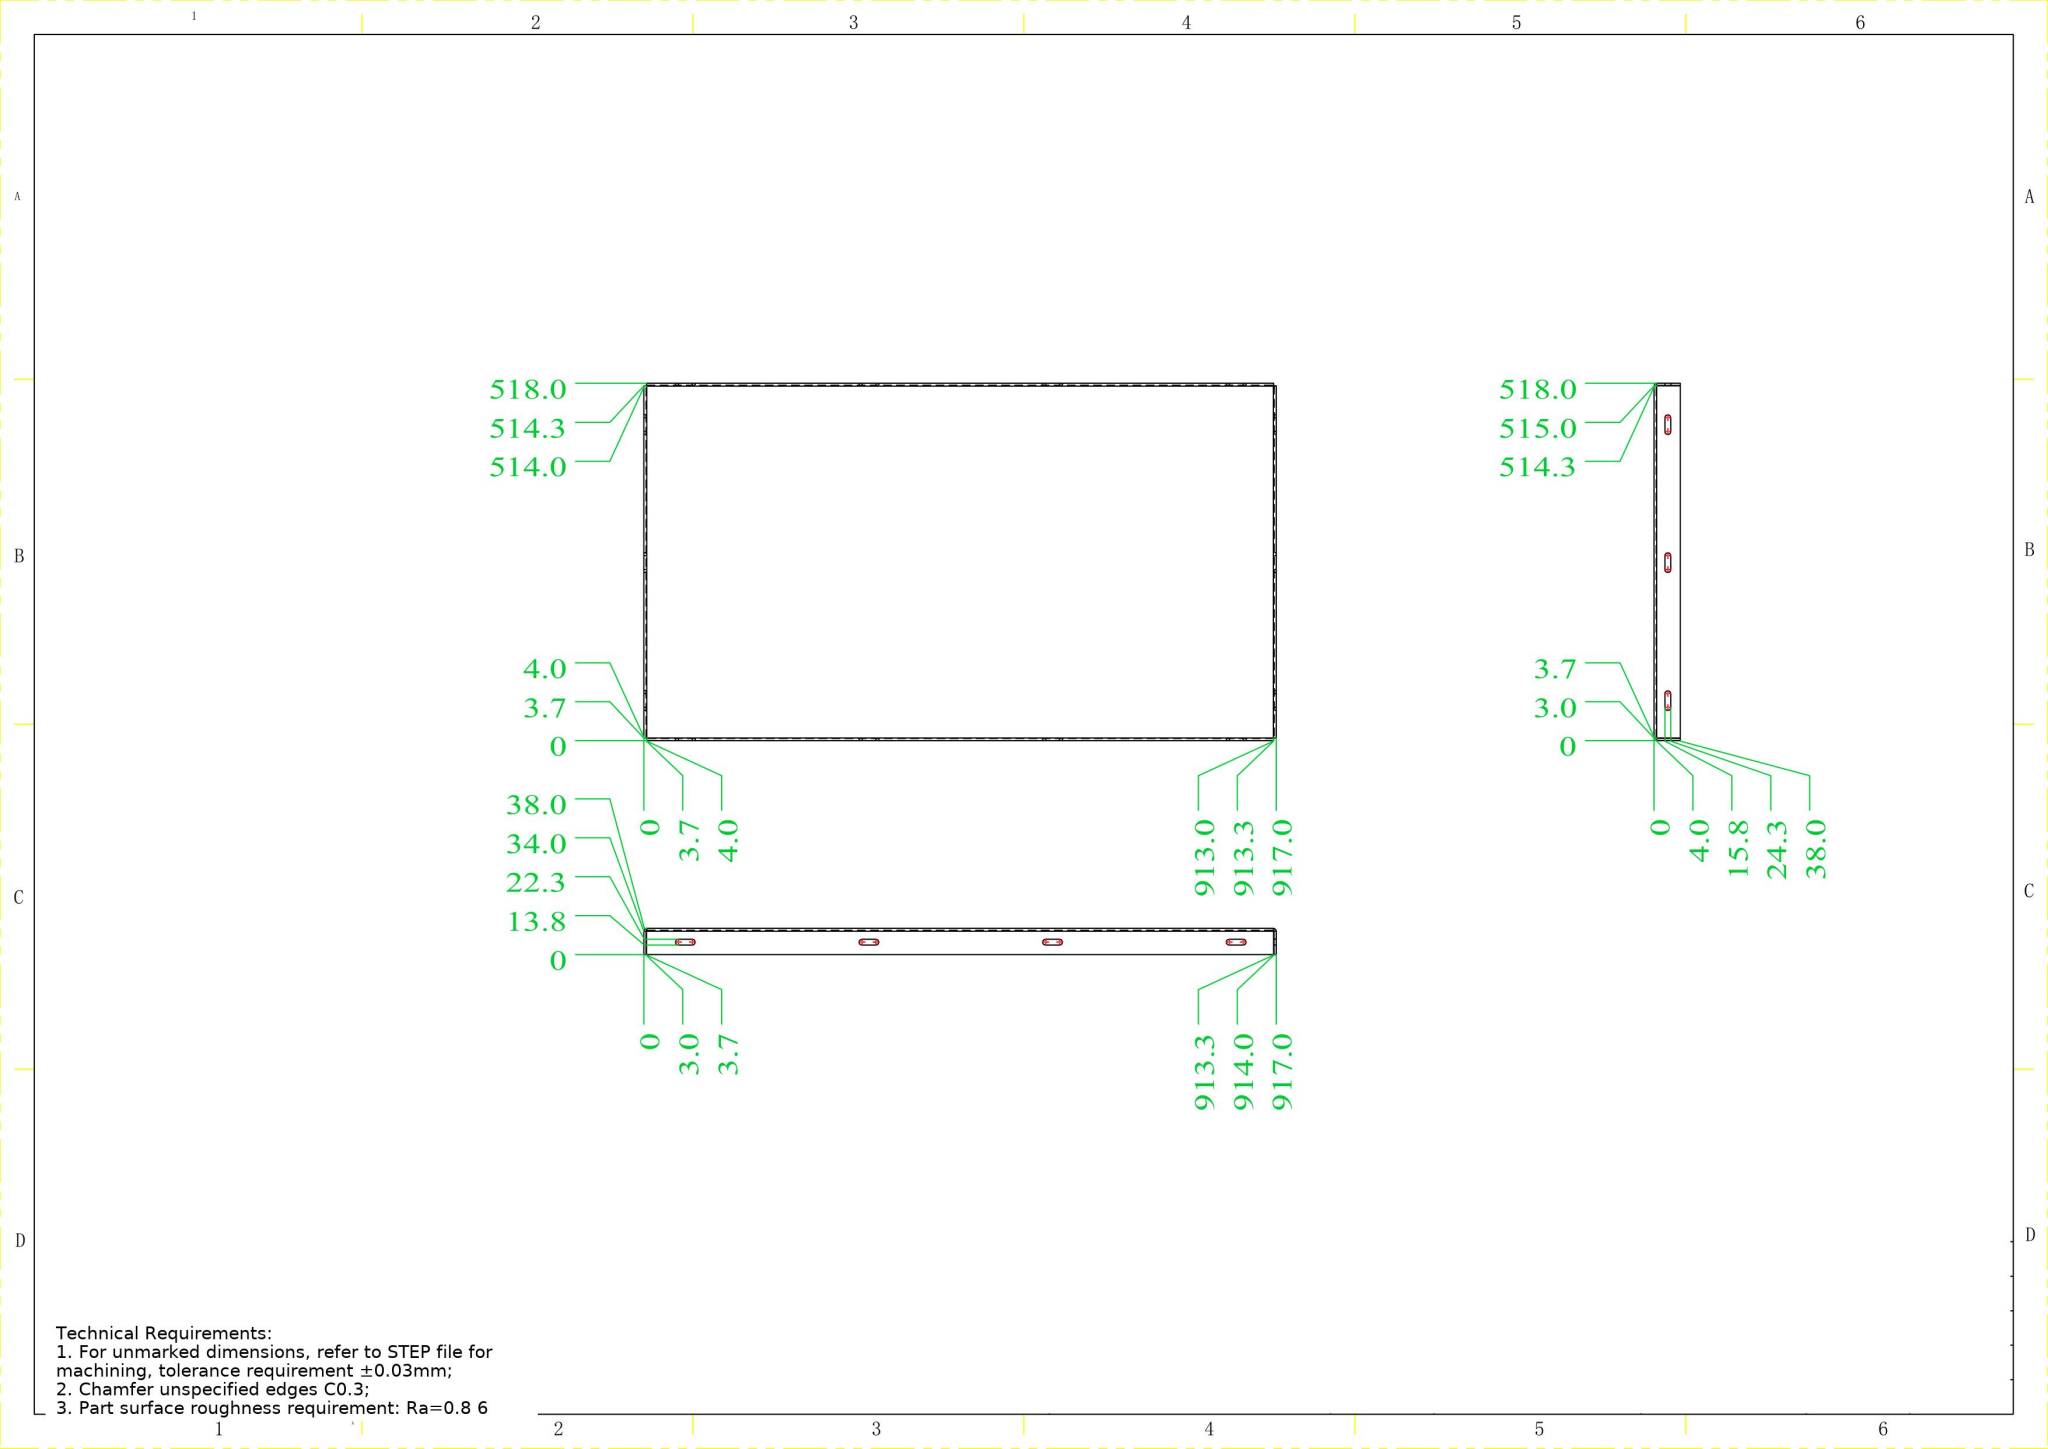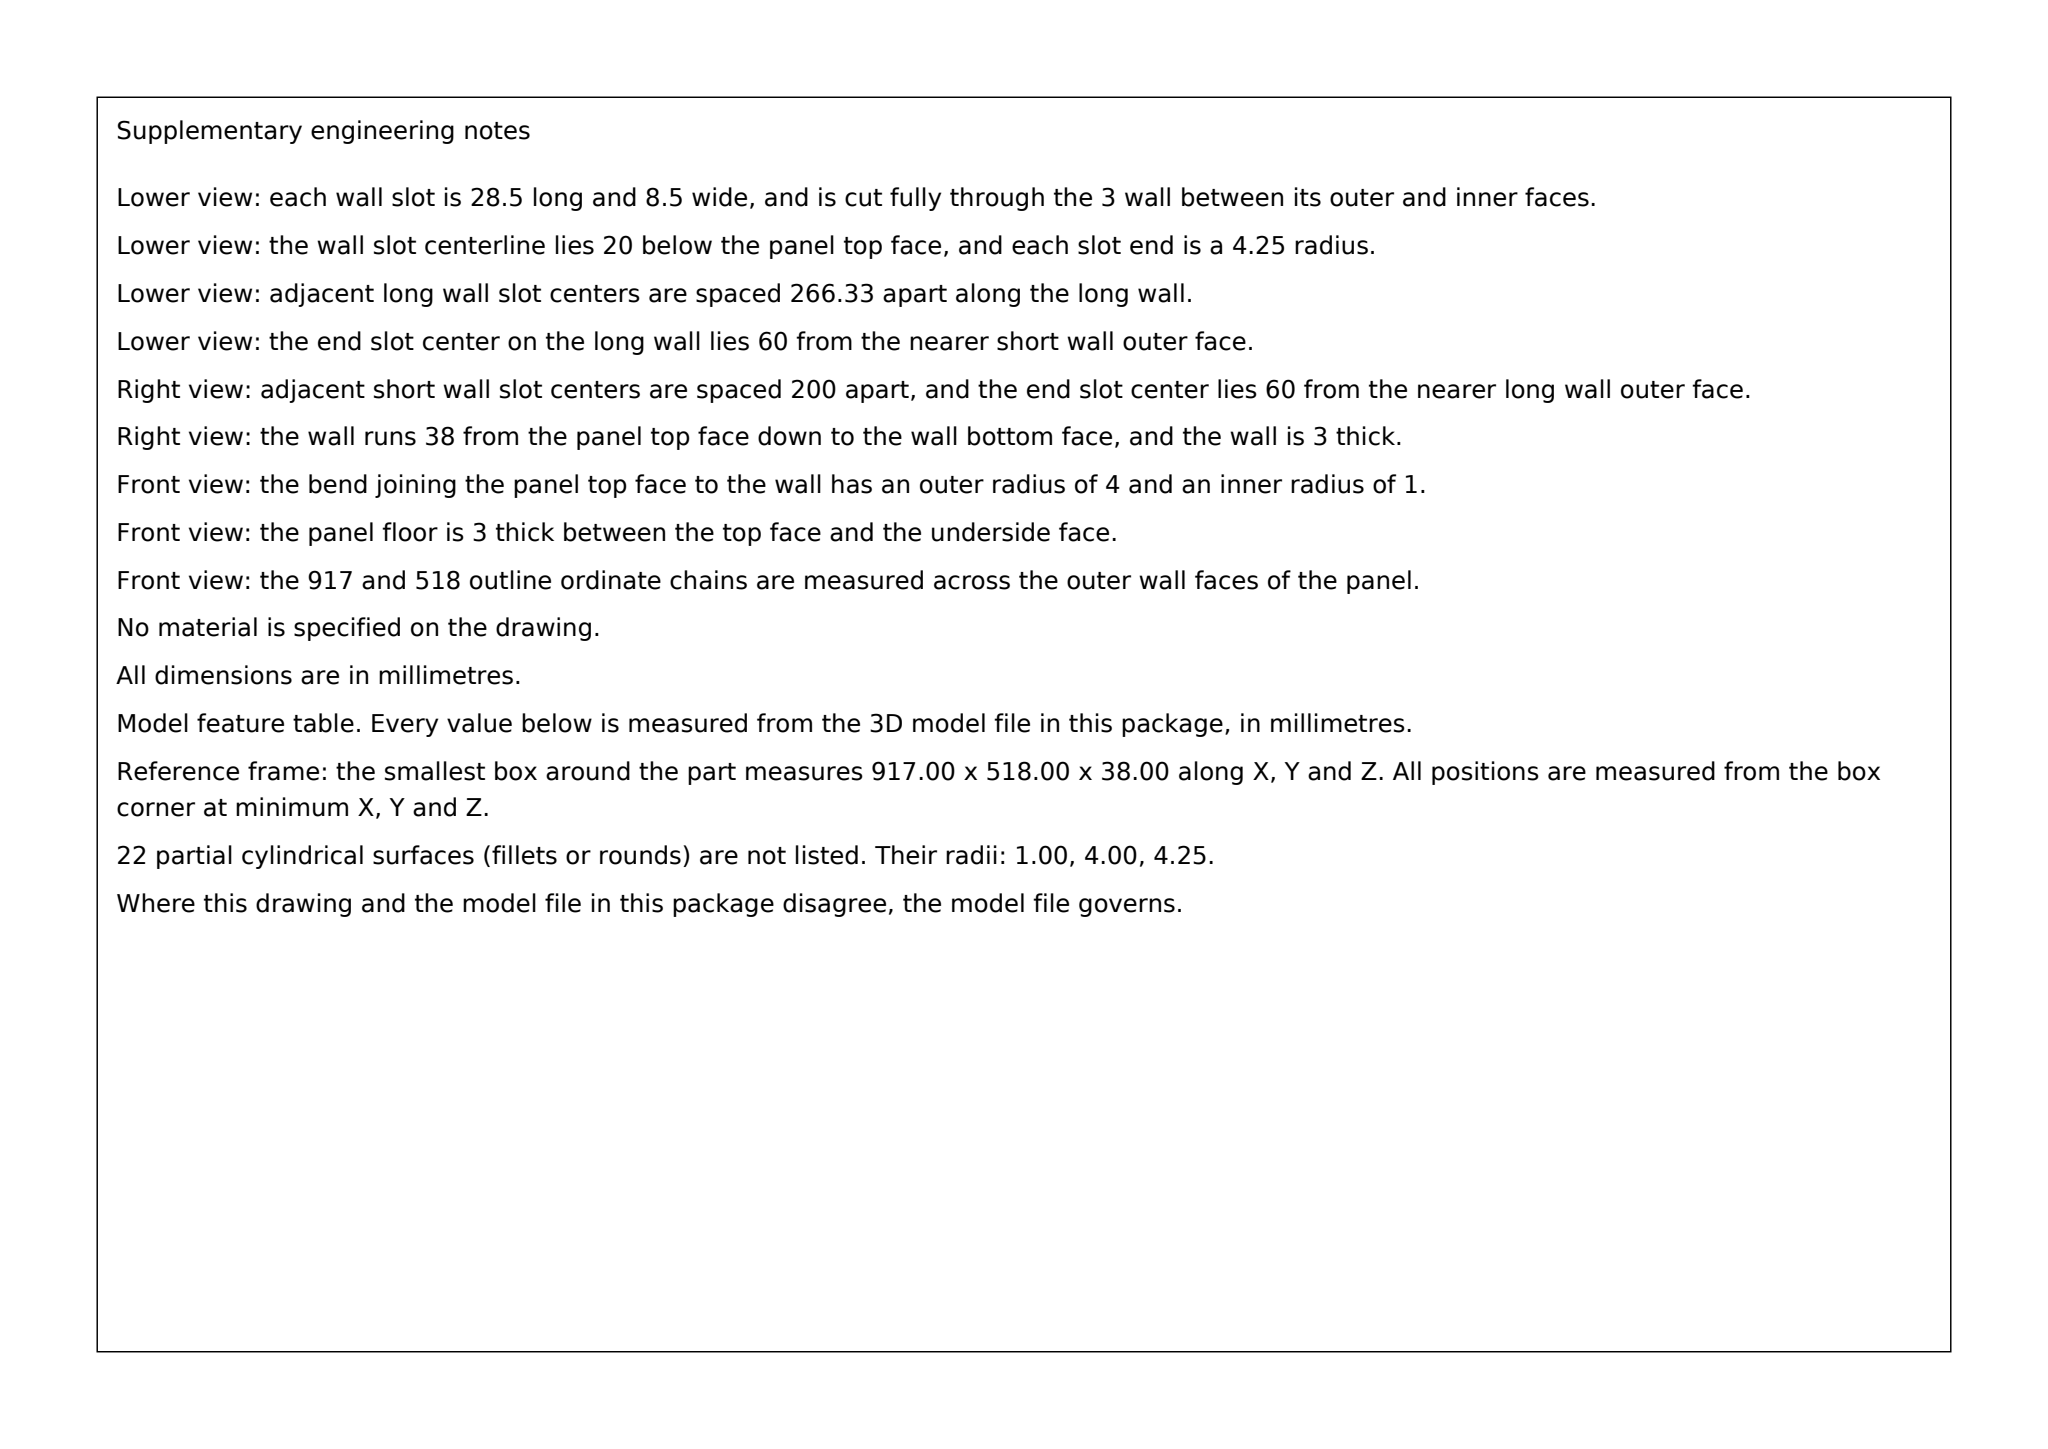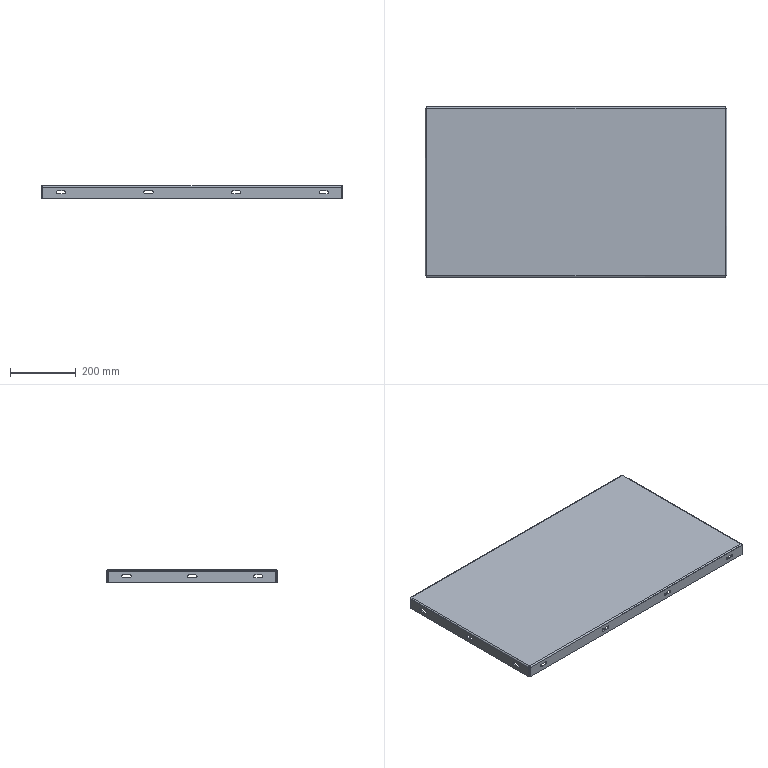Part | SolidWorks | mm | 1 solid | 94 faces | box 917 x 518 x 38 mm | volume 1704410 mm3 | plane 50 | cylinder 36 | spline 8 | commonest cylinder face diameters 8.5 x28 8 x4 2 x4
Drawing notes:
14X 8.5 WIDE OBROUND SLOT, 28.5 OVERALL LENGTH (20.0 BETWEEN END-RADII CENTERS), THRU 3.0 WALL, SLOT CENTERLINE AT Z=18.0 FROM BOTTOM FACE | from the solid: cylinders dia 8.5, length 3.0, pos z=18.0; paired centers 20 mm apart (e.g. y=48.03 & 68.03; x=50.03 & 70.03)
SLOTS IN EACH 917 LONG WALL (8 PLACES, 4 PER WALL): END-RADII CENTERS AT X=50.0 & 70.0, 316.4 & 336.4, 582.7 & 602.7, 849.0 & 869.0 FROM X=0 DATUM | from the solid: cylinders[8.5,"y",[50.03/70.03/316.36/336.36/582.69/602.69/849.02/869.02,null,18.0],3.0,2]
SLOTS IN EACH 518 END WALL (6 PLACES, 3 PER WALL): END-RADII CENTERS AT Y=48.0 & 68.0, 248.0 & 268.0, 448.0 & 468.0 FROM Y=0 DATUM | from the solid: cylinders[8.5,"x",[null,48.03/68.03/248.03/268.03/448.03/468.03,18.0],3.0,2]
PATTERN: 4X SLOTS TYP EACH 917 SIDE, 3X SLOTS TYP EACH 518 SIDE, 14 SLOTS TOTAL | from the solid: cylinders dia 8.5 axis y: 8 pair-entries count 2 (4 slots x 2 walls); axis x: 6 pair-entries count 2 (3 slots x 2 walls)
Ø8 INTERNAL LONGITUDINAL BORE AT Z=34.0, AXIS 4.0 FROM OUTSIDE FACE: 2X 909.6 LONG ALONG THE 917 EDGES (Y=4.0 AND Y=514.0), 2X 510.6 LONG ALONG THE 518 EDGES (X=4.0 AND X=913.0) | from the solid: cylinders[8.0,"x",[null,4.03/514.03,34.0],909.59] and cylinders[8.0,"y",[4.03/913.03,null,34.0],510.59]
Ø2 OPENING SLIT INTO EACH Ø8 LONGITUDINAL BORE, COAXIAL AT Z=34.0 AND 4.0 FROM OUTSIDE FACE, 4 PLACES, SAME LENGTHS AS BORES (909.6 / 510.6) | from the solid: cylinders[2.0,"x",[null,4.03/514.03,34.0],909.59] and cylinders[2.0,"y",[4.03/913.03,null,34.0],510.59]
STEP AT TOP OF WALLS: FACE AT Z=35.0, 3.0 BELOW THE Z=38.0 TOP FACE (38.0 OVERALL HEIGHT FROM Z=0 BOTTOM DATUM); STEP FACE BOUNDED BY X=3.0 TO 914.0 AND Y=3.0 TO 515.0 FROM X=0 / Y=0 DATUMS | from the solid: axis_planes z offset 35.0 (count 1) and z offset 38.0 (count 1), bbox_xyz Z=38.03; bounding planes x 3.03 & 914.03, y 3.03 & 515.03